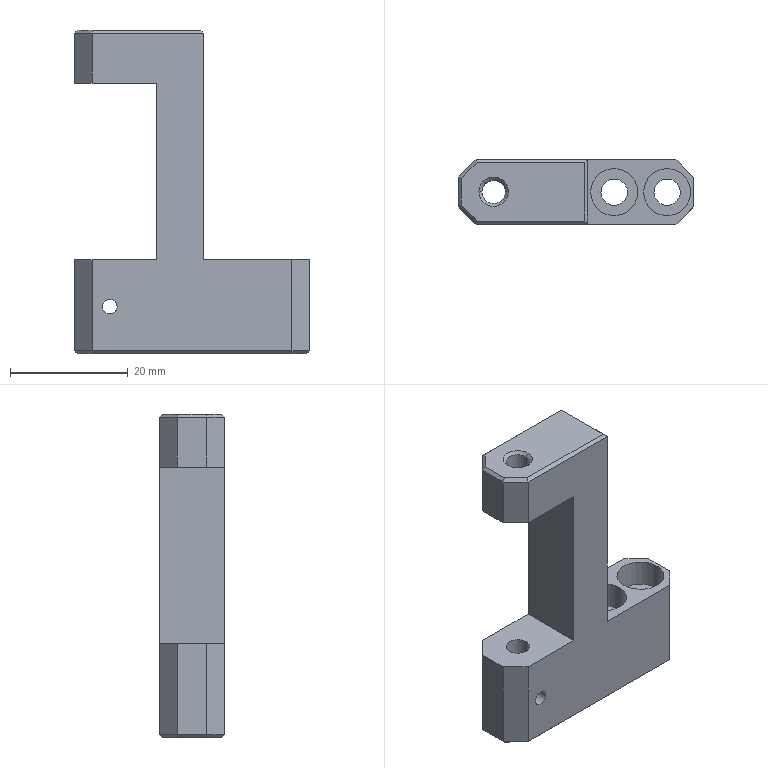Component | SolidWorks | LowerRollerMountingSeat-1 | 1 solid | 58 faces | volume 10288 mm3 | plane 34 | cylinder 16 | cone 8 | commonest cylinder face diameters 2.5 x4 4 x4 8 x4 4.5 x4